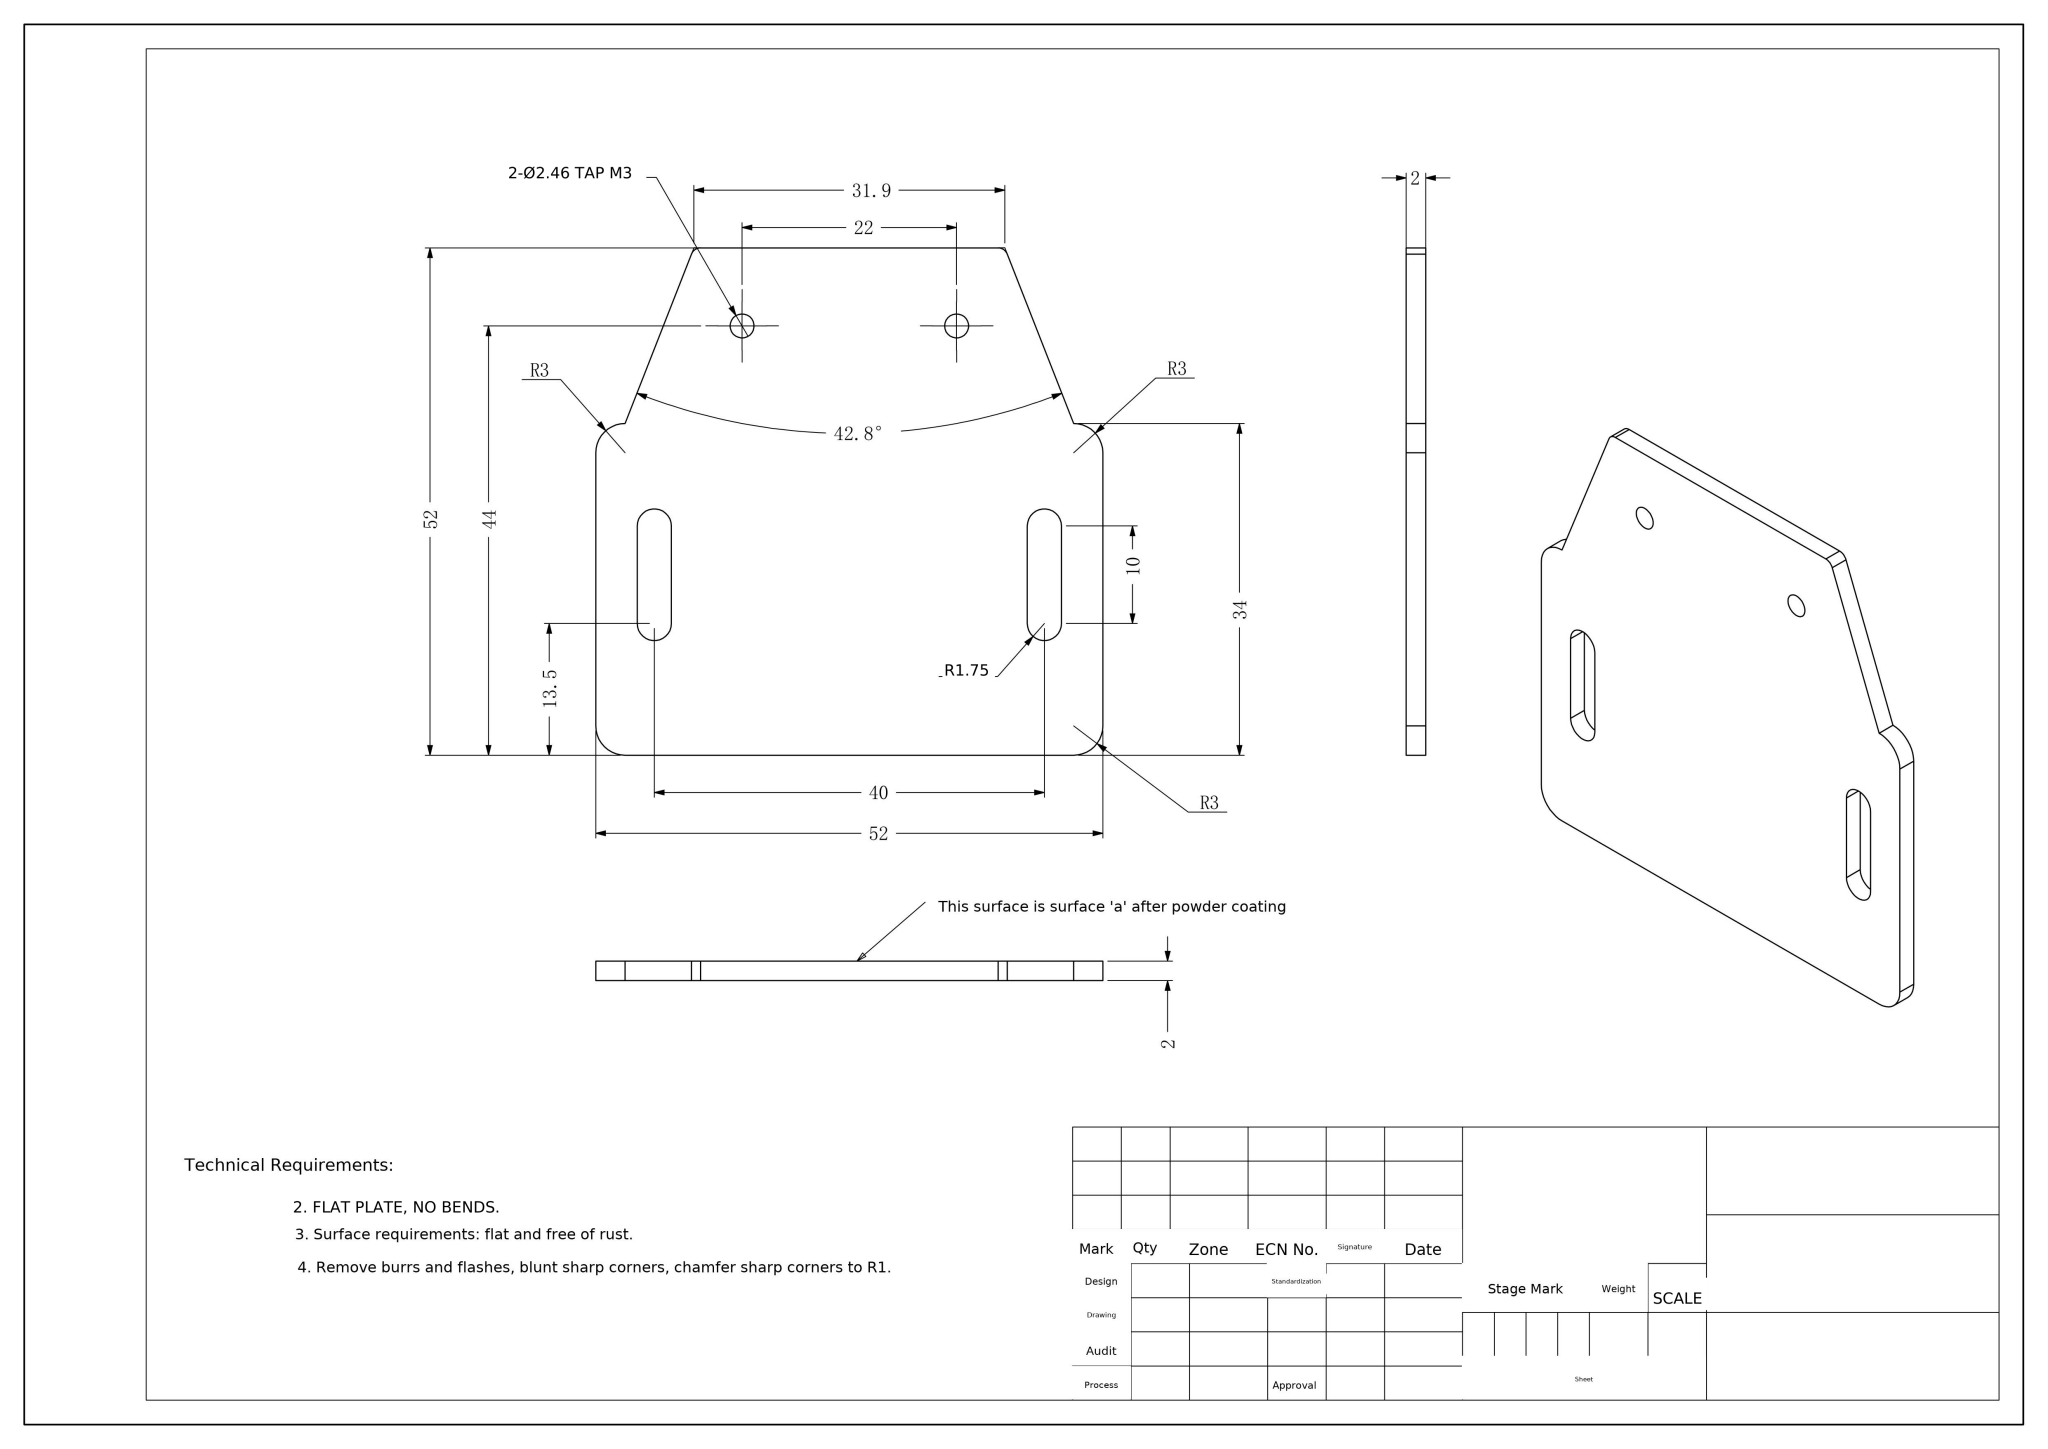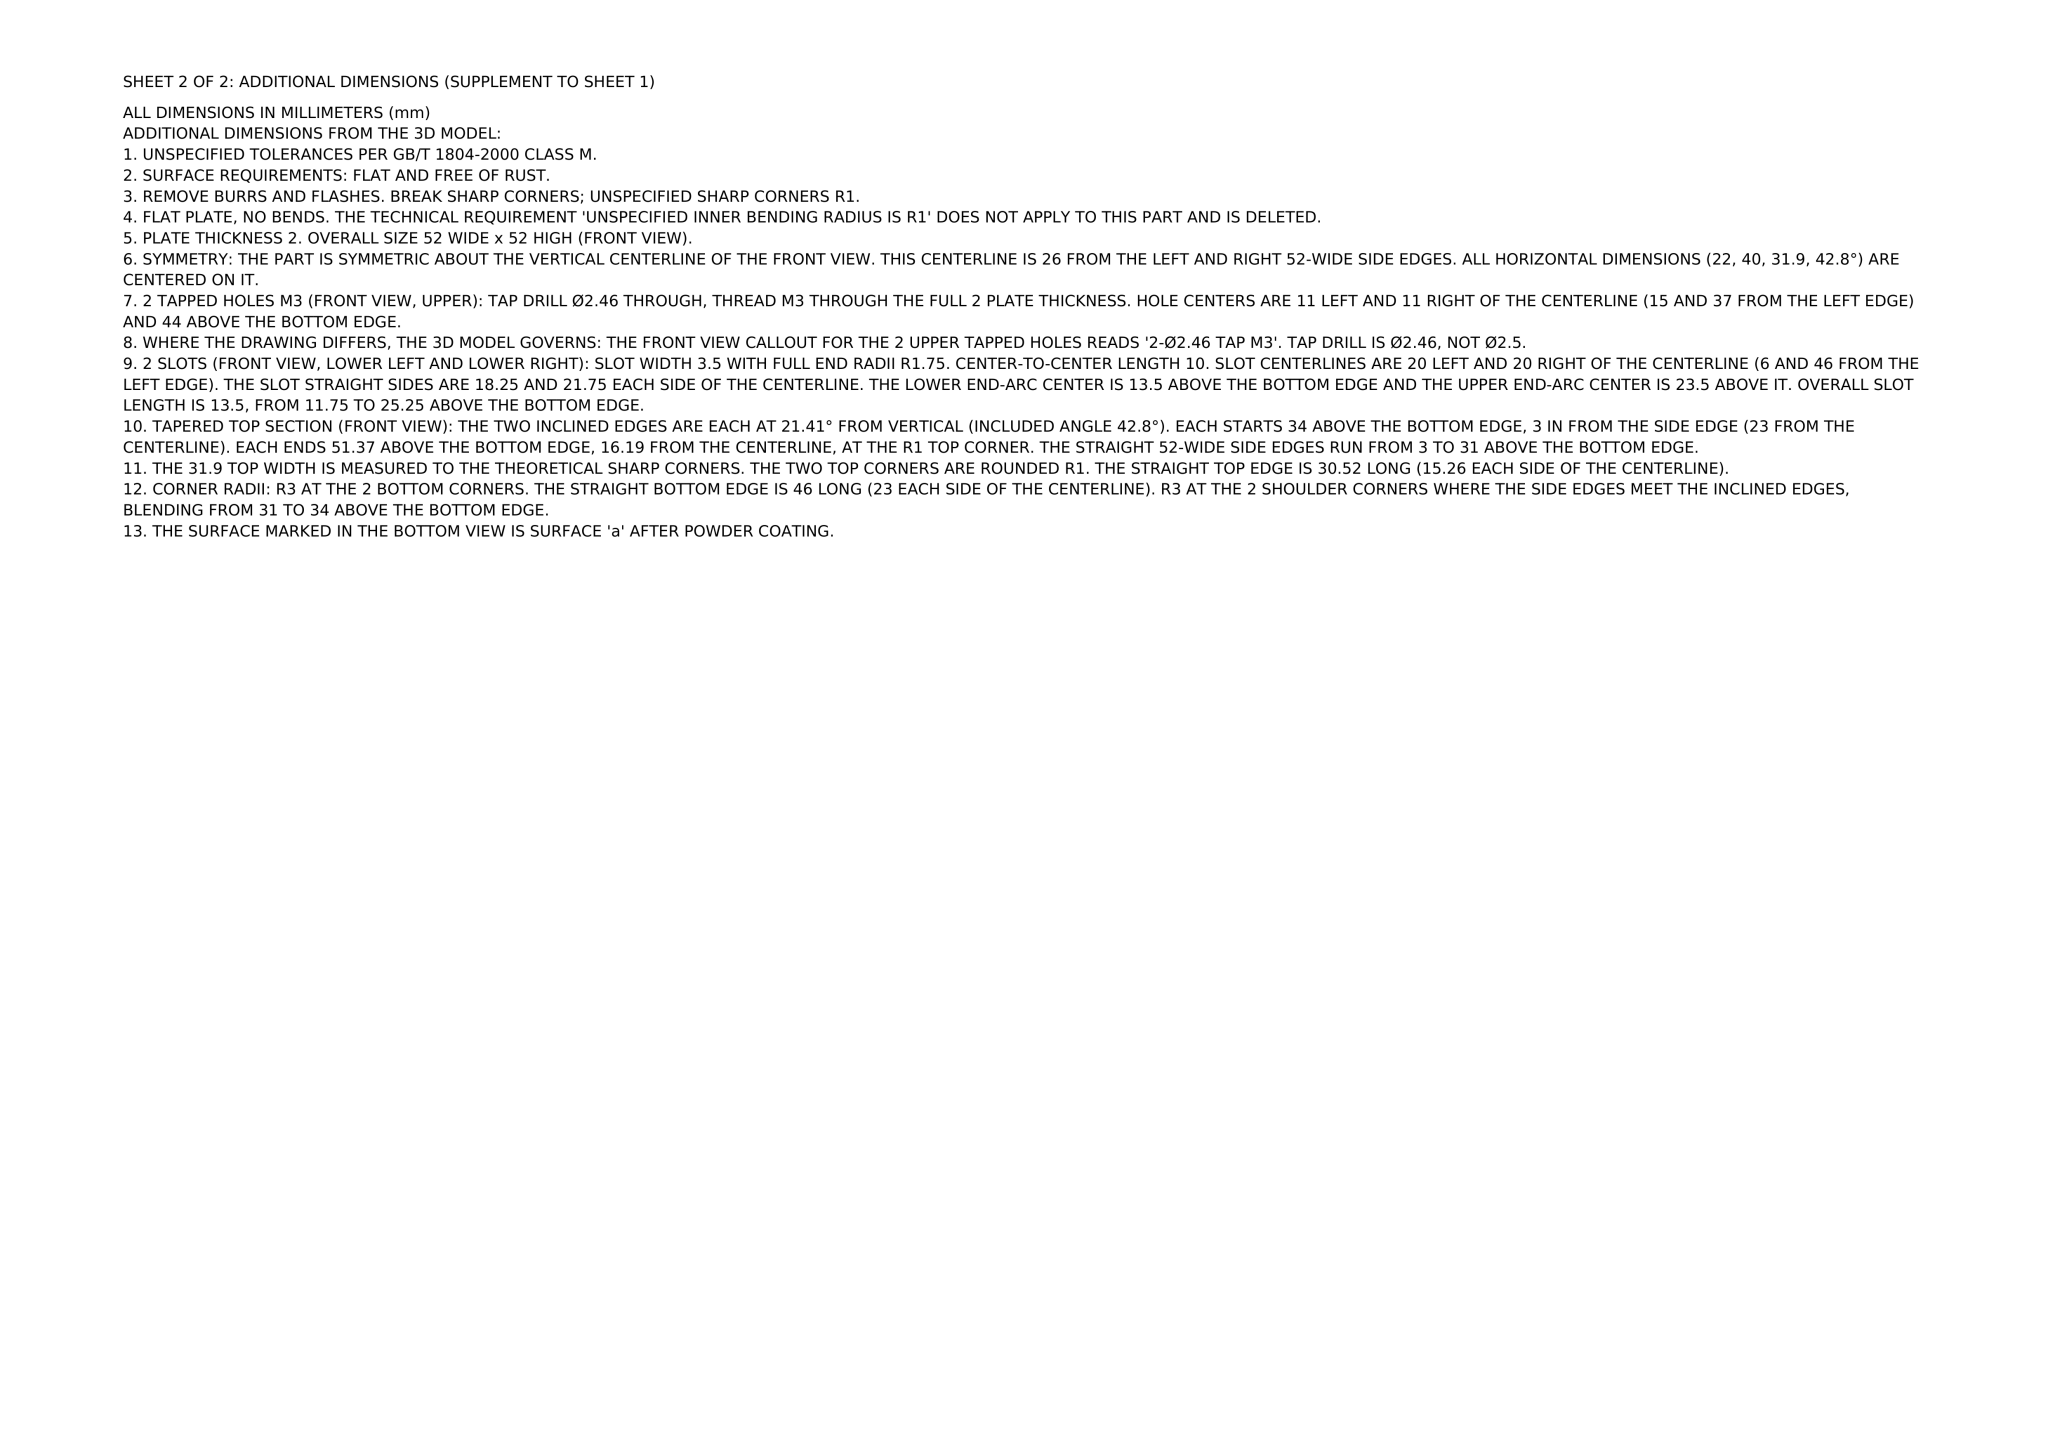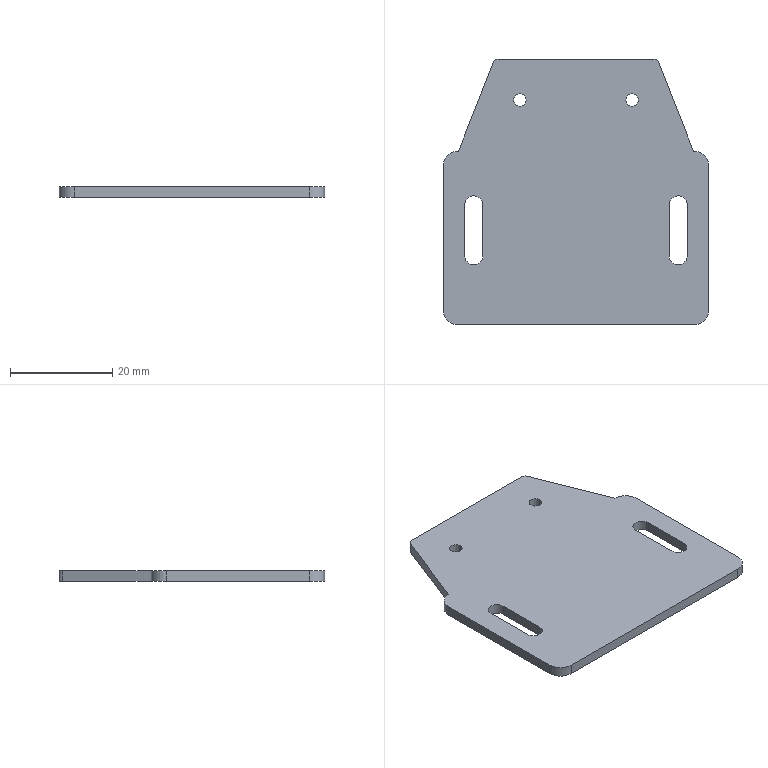Part | NX | mm | Tapered Edge Dual-Slot Mounting Plate | 1 solid | 26 faces | box 52 x 52 x 2 mm | volume 4725 mm3 | cylinder 14 | plane 12 | commonest cylinder face diameters 2.459 x4 6 x4 3.5 x4 2 x2